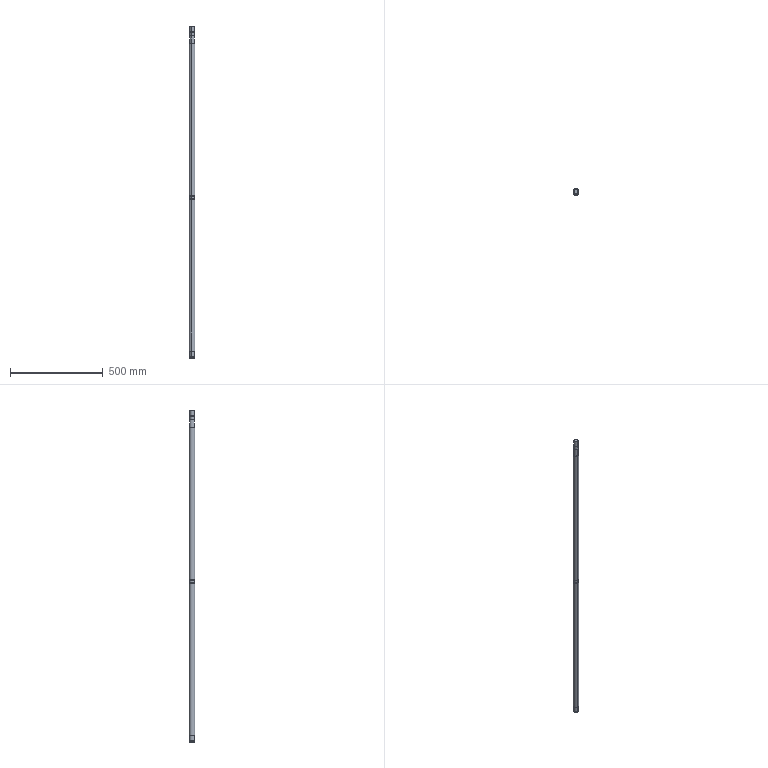Component | SolidWorks | R32-6B2-FSW-331-1 | 1 solid | 44 faces | box 32 x 32 x 1785 mm | volume 1385317 mm3 | cylinder 18 | cone 14 | plane 10 | torus 2 | commonest cylinder face diameters 25 x6 32 x4 23.8 x2 26 x2 23.376 x2 22 x2 | material Plain Carbon Steel
build123d program:
from build123d import *

# Parameters (mm, degrees)
CHAMFER1_SIZE = 1
CHAMFER3_SIZE = 0.5
FILLET1_R     = 0.5
CHAMFER4_SIZE = 1


with BuildPart() as part:
    # Sketch1 → Revolve1 (revolve)
    with BuildSketch(Plane.XY, mode=Mode.PRIVATE) as revolve1_sk:
        Polygon((0, 0), (0, 11), (32, 11), (32, 11.688), (52, 11.688), (52, 12.5), (95, 12.5), (95, 16), (915, 16), (915, 13), (930, 13), (930, 16), (1749, 16), (1749, 12.5), (1779, 12.5), (1779, 11.9), (1780.35, 11.9), (1780.35, 12.5), (1785, 12.5), (1785, 0), align=None)
    revolve(revolve1_sk.sketch.rotate(Axis((-159.723, 0, 0), (1, 0, 0)), 180), axis=Axis((-159.723, 0, 0), (1, 0, 0)))

    # Chamfer1
    chamfer1_edges = [part.edges().sort_by_distance(p)[0] for p in [
        (0, 11, 0),
    ]]
    chamfer(chamfer1_edges, length=CHAMFER1_SIZE)

    # Chamfer3
    chamfer3_edges = [part.edges().sort_by_distance(p)[0] for p in [
        (32, 11.688, 0),
    ]]
    chamfer(chamfer3_edges, length=CHAMFER3_SIZE)

    # Fillet1
    fillet1_edges = [part.edges().sort_by_distance(p)[0] for p in [
        (95, 12.5, 0),
    ]]
    fillet(fillet1_edges, radius=FILLET1_R)

    # Chamfer4
    chamfer4_edges = [part.edges().sort_by_distance(p)[0] for p in [
        (1785, 12.5, 0),
        (1749, 16, 0),
        (930, 16, 0),
        (915, 16, 0),
        (95, 16, 0),
    ]]
    chamfer(chamfer4_edges, length=CHAMFER4_SIZE)


solid = part.part

# Placed as in the assembly
solid = solid.moved(Location((5.881, 3.444, 63.5), (0, 90, 0)))